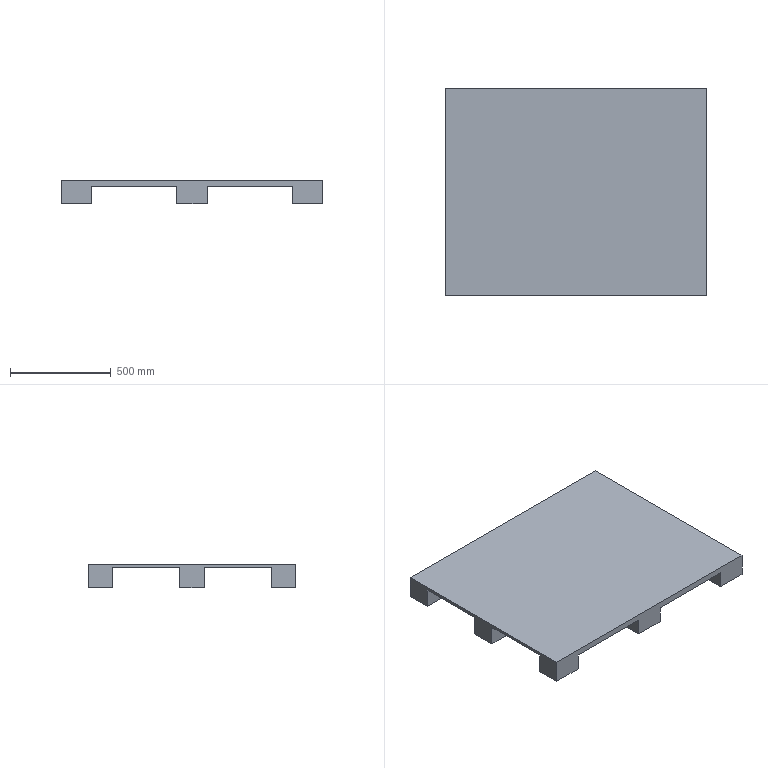Component | NX | 103X135X10_PALLET | 1 solid | 38 faces | volume 40875000 mm3 | plane 38